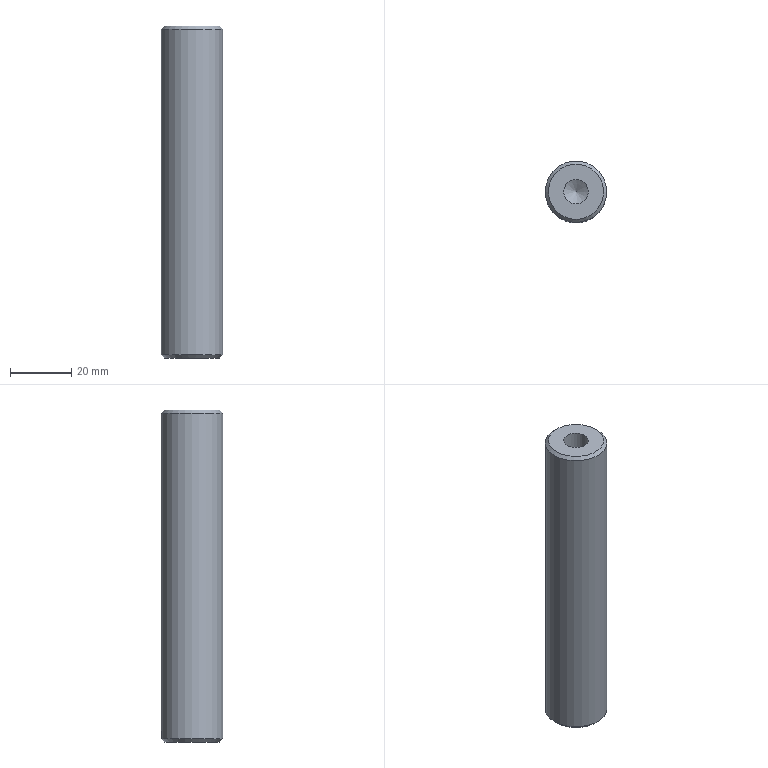Component | NX | GUIDE_POST | 1 solid | 9 faces | box 20 x 20 x 108 mm | volume 32179 mm3 | cone 4 | cylinder 3 | plane 2 | commonest cylinder face diameters 8 x2 20 x1
STEP:
#1=CARTESIAN_POINT('',(0.,0.,0.));
#2=DIRECTION('',(0.,0.,1.));
#3=DIRECTION('',(1.,0.,0.));
#4=AXIS2_PLACEMENT_3D('',#1,#2,#3);
#5=CARTESIAN_POINT('',(-177.087,-60.,105.));
#6=VERTEX_POINT('',#5);
#7=CARTESIAN_POINT('',(-186.087,-60.,105.));
#8=DIRECTION('',(0.,0.,1.));
#9=DIRECTION('',(1.,0.,0.));
#10=AXIS2_PLACEMENT_3D('',#7,#8,#9);
#11=CIRCLE('',#10,9.);
#12=CARTESIAN_POINT('',(-186.087,-60.,105.));
#13=DIRECTION('',(0.,0.,1.));
#14=DIRECTION('',(1.,0.,0.));
#15=AXIS2_PLACEMENT_3D('',#12,#13,#14);
#16=PLANE('',#15);
#17=CARTESIAN_POINT('',(0.,0.));
#18=DIRECTION('',(1.,0.));
#19=AXIS2_PLACEMENT_2D('',#17,#18);
#20=CIRCLE('',#19,9.);
#21=(GEOMETRIC_REPRESENTATION_CONTEXT(2)PARAMETRIC_REPRESENTATION_CONTEXT()REPRESENTATION_CONTEXT('',''));
#22=DEFINITIONAL_REPRESENTATION('',(#20),#21);
#23=PCURVE('',#16,#22);
#24=CARTESIAN_POINT('',(-186.087,-60.,104.));
#25=DIRECTION('',(0.,0.,-1.));
#26=DIRECTION('',(-1.,0.,0.));
#27=AXIS2_PLACEMENT_3D('',#24,#25,#26);
#28=CONICAL_SURFACE('',#27,10.,0.7854);
#29=CARTESIAN_POINT('',(9.425,-1.));
#30=DIRECTION('',(-1.,0.));
#31=VECTOR('',#30,1.);
#32=LINE('',#29,#31);
#33=(GEOMETRIC_REPRESENTATION_CONTEXT(2)PARAMETRIC_REPRESENTATION_CONTEXT()REPRESENTATION_CONTEXT('',''));
#34=DEFINITIONAL_REPRESENTATION('',(#32),#33);
#35=PCURVE('',#28,#34);
#36=SURFACE_CURVE('',#11,(#23,#35),.PCURVE_S1.);
#37=EDGE_CURVE('',#6,#6,#36,.T.);
#38=ORIENTED_EDGE('',*,*,#37,.T.);
#39=EDGE_LOOP('',(#38));
#40=FACE_BOUND('',#39,.T.);
#41=CARTESIAN_POINT('',(-190.087,-60.,105.));
#42=VERTEX_POINT('',#41);
#43=CARTESIAN_POINT('',(-186.087,-60.,105.));
#44=DIRECTION('',(0.,0.,-1.));
#45=DIRECTION('',(-1.,0.,0.));
#46=AXIS2_PLACEMENT_3D('',#43,#44,#45);
#47=CIRCLE('',#46,4.);
#48=CARTESIAN_POINT('',(-4.,0.));
#49=CARTESIAN_POINT('',(-4.,6.928));
#50=CARTESIAN_POINT('',(2.,3.464));
#51=CARTESIAN_POINT('',(8.,0.));
#52=CARTESIAN_POINT('',(2.,-3.464));
#53=CARTESIAN_POINT('',(-4.,-6.928));
#54=CARTESIAN_POINT('',(-4.,0.));
#55=(BOUNDED_CURVE()B_SPLINE_CURVE(2,(#48,#49,#50,#51,#52,#53,#54),.UNSPECIFIED.,.T.,.F.)B_SPLINE_CURVE_WITH_KNOTS((1,2,2,2,2,1),(-2.094,0.,2.094,4.189,6.283,8.378),.UNSPECIFIED.)CURVE()GEOMETRIC_REPRESENTATION_ITEM()RATIONAL_B_SPLINE_CURVE((1.,0.5,1.,0.5,1.,0.5,1.))REPRESENTATION_ITEM(''));
#56=(GEOMETRIC_REPRESENTATION_CONTEXT(2)PARAMETRIC_REPRESENTATION_CONTEXT()REPRESENTATION_CONTEXT('',''));
#57=DEFINITIONAL_REPRESENTATION('',(#55),#56);
#58=PCURVE('',#16,#57);
#59=CARTESIAN_POINT('',(-186.087,-60.,105.));
#60=DIRECTION('',(0.,0.,-1.));
#61=DIRECTION('',(-1.,0.,0.));
#62=AXIS2_PLACEMENT_3D('',#59,#60,#61);
#63=CYLINDRICAL_SURFACE('',#62,4.);
#64=CARTESIAN_POINT('',(0.,0.));
#65=DIRECTION('',(1.,0.));
#66=VECTOR('',#65,1.);
#67=LINE('',#64,#66);
#68=(GEOMETRIC_REPRESENTATION_CONTEXT(2)PARAMETRIC_REPRESENTATION_CONTEXT()REPRESENTATION_CONTEXT('',''));
#69=DEFINITIONAL_REPRESENTATION('',(#67),#68);
#70=PCURVE('',#63,#69);
#71=SURFACE_CURVE('',#47,(#58,#70),.PCURVE_S1.);
#72=EDGE_CURVE('',#42,#42,#71,.T.);
#73=ORIENTED_EDGE('',*,*,#72,.T.);
#74=EDGE_LOOP('',(#73));
#75=FACE_BOUND('',#74,.T.);
#76=ADVANCED_FACE('',(#40,#75),#16,.T.);
#77=CARTESIAN_POINT('',(-195.087,-60.,-3.));
#78=VERTEX_POINT('',#77);
#79=CARTESIAN_POINT('',(-186.087,-60.,-3.));
#80=DIRECTION('',(0.,0.,-1.));
#81=DIRECTION('',(-1.,0.,0.));
#82=AXIS2_PLACEMENT_3D('',#79,#80,#81);
#83=CIRCLE('',#82,9.);
#84=CARTESIAN_POINT('',(-186.087,-60.,-3.));
#85=DIRECTION('',(0.,0.,-1.));
#86=DIRECTION('',(-1.,0.,0.));
#87=AXIS2_PLACEMENT_3D('',#84,#85,#86);
#88=PLANE('',#87);
#89=CARTESIAN_POINT('',(0.,0.));
#90=DIRECTION('',(1.,0.));
#91=AXIS2_PLACEMENT_2D('',#89,#90);
#92=CIRCLE('',#91,9.);
#93=(GEOMETRIC_REPRESENTATION_CONTEXT(2)PARAMETRIC_REPRESENTATION_CONTEXT()REPRESENTATION_CONTEXT('',''));
#94=DEFINITIONAL_REPRESENTATION('',(#92),#93);
#95=PCURVE('',#88,#94);
#96=CARTESIAN_POINT('',(-186.087,-60.,-2.));
#97=DIRECTION('',(0.,0.,1.));
#98=DIRECTION('',(1.,0.,0.));
#99=AXIS2_PLACEMENT_3D('',#96,#97,#98);
#100=CONICAL_SURFACE('',#99,10.,0.7854);
#101=CARTESIAN_POINT('',(9.425,-1.));
#102=DIRECTION('',(-1.,0.));
#103=VECTOR('',#102,1.);
#104=LINE('',#101,#103);
#105=(GEOMETRIC_REPRESENTATION_CONTEXT(2)PARAMETRIC_REPRESENTATION_CONTEXT()REPRESENTATION_CONTEXT('',''));
#106=DEFINITIONAL_REPRESENTATION('',(#104),#105);
#107=PCURVE('',#100,#106);
#108=SURFACE_CURVE('',#83,(#95,#107),.PCURVE_S1.);
#109=EDGE_CURVE('',#78,#78,#108,.T.);
#110=ORIENTED_EDGE('',*,*,#109,.T.);
#111=EDGE_LOOP('',(#110));
#112=FACE_BOUND('',#111,.T.);
#113=CARTESIAN_POINT('',(-182.087,-60.,-3.));
#114=VERTEX_POINT('',#113);
#115=CARTESIAN_POINT('',(-186.087,-60.,-3.));
#116=DIRECTION('',(0.,0.,1.));
#117=DIRECTION('',(1.,0.,0.));
#118=AXIS2_PLACEMENT_3D('',#115,#116,#117);
#119=CIRCLE('',#118,4.);
#120=CARTESIAN_POINT('',(-4.,0.));
#121=CARTESIAN_POINT('',(-4.,6.928));
#122=CARTESIAN_POINT('',(2.,3.464));
#123=CARTESIAN_POINT('',(8.,0.));
#124=CARTESIAN_POINT('',(2.,-3.464));
#125=CARTESIAN_POINT('',(-4.,-6.928));
#126=CARTESIAN_POINT('',(-4.,0.));
#127=(BOUNDED_CURVE()B_SPLINE_CURVE(2,(#120,#121,#122,#123,#124,#125,#126),.UNSPECIFIED.,.T.,.F.)B_SPLINE_CURVE_WITH_KNOTS((1,2,2,2,2,1),(-2.094,0.,2.094,4.189,6.283,8.378),.UNSPECIFIED.)CURVE()GEOMETRIC_REPRESENTATION_ITEM()RATIONAL_B_SPLINE_CURVE((1.,0.5,1.,0.5,1.,0.5,1.))REPRESENTATION_ITEM(''));
#128=(GEOMETRIC_REPRESENTATION_CONTEXT(2)PARAMETRIC_REPRESENTATION_CONTEXT()REPRESENTATION_CONTEXT('',''));
#129=DEFINITIONAL_REPRESENTATION('',(#127),#128);
#130=PCURVE('',#88,#129);
#131=CARTESIAN_POINT('',(-186.087,-60.,-3.));
#132=DIRECTION('',(0.,0.,1.));
#133=DIRECTION('',(1.,0.,0.));
#134=AXIS2_PLACEMENT_3D('',#131,#132,#133);
#135=CYLINDRICAL_SURFACE('',#134,4.);
#136=CARTESIAN_POINT('',(0.,0.));
#137=DIRECTION('',(1.,0.));
#138=VECTOR('',#137,1.);
#139=LINE('',#136,#138);
#140=(GEOMETRIC_REPRESENTATION_CONTEXT(2)PARAMETRIC_REPRESENTATION_CONTEXT()REPRESENTATION_CONTEXT('',''));
#141=DEFINITIONAL_REPRESENTATION('',(#139),#140);
#142=PCURVE('',#135,#141);
#143=SURFACE_CURVE('',#119,(#130,#142),.PCURVE_S1.);
#144=EDGE_CURVE('',#114,#114,#143,.T.);
#145=ORIENTED_EDGE('',*,*,#144,.T.);
#146=EDGE_LOOP('',(#145));
#147=FACE_BOUND('',#146,.T.);
#148=ADVANCED_FACE('',(#112,#147),#88,.T.);
#149=CARTESIAN_POINT('',(-196.087,-60.,-2.));
#150=VERTEX_POINT('',#149);
#151=CARTESIAN_POINT('',(-176.087,-60.,-2.));
#152=VERTEX_POINT('',#151);
#153=CARTESIAN_POINT('',(-186.087,-60.,-2.));
#154=DIRECTION('',(0.,0.,1.));
#155=DIRECTION('',(-1.,0.,0.));
#156=AXIS2_PLACEMENT_3D('',#153,#154,#155);
#157=CIRCLE('',#156,10.);
#158=CARTESIAN_POINT('',(-186.087,-60.,-3.));
#159=DIRECTION('',(0.,0.,1.));
#160=DIRECTION('',(1.,0.,0.));
#161=AXIS2_PLACEMENT_3D('',#158,#159,#160);
#162=CYLINDRICAL_SURFACE('',#161,10.);
#163=CARTESIAN_POINT('',(3.142,1.));
#164=DIRECTION('',(1.,0.));
#165=VECTOR('',#164,1.);
#166=LINE('',#163,#165);
#167=(GEOMETRIC_REPRESENTATION_CONTEXT(2)PARAMETRIC_REPRESENTATION_CONTEXT()REPRESENTATION_CONTEXT('',''));
#168=DEFINITIONAL_REPRESENTATION('',(#166),#167);
#169=PCURVE('',#162,#168);
#170=CARTESIAN_POINT('',(3.142,0.));
#171=DIRECTION('',(1.,0.));
#172=VECTOR('',#171,1.);
#173=LINE('',#170,#172);
#174=(GEOMETRIC_REPRESENTATION_CONTEXT(2)PARAMETRIC_REPRESENTATION_CONTEXT()REPRESENTATION_CONTEXT('',''));
#175=DEFINITIONAL_REPRESENTATION('',(#173),#174);
#176=PCURVE('',#100,#175);
#177=SURFACE_CURVE('',#157,(#169,#176),.PCURVE_S1.);
#178=EDGE_CURVE('',#150,#152,#177,.T.);
#179=ORIENTED_EDGE('',*,*,#178,.T.);
#180=CARTESIAN_POINT('',(-176.087,-60.,104.));
#181=VERTEX_POINT('',#180);
#182=CARTESIAN_POINT('',(-176.087,-60.,-2.));
#183=CARTESIAN_POINT('',(-176.087,-60.,104.));
#184=B_SPLINE_CURVE_WITH_KNOTS('',1,(#182,#183),.UNSPECIFIED.,.F.,.F.,(2,2),(1.,107.),.PIECEWISE_BEZIER_KNOTS.);
#185=CARTESIAN_POINT('',(6.283,0.));
#186=DIRECTION('',(0.,1.));
#187=VECTOR('',#186,1.);
#188=LINE('',#185,#187);
#189=(GEOMETRIC_REPRESENTATION_CONTEXT(2)PARAMETRIC_REPRESENTATION_CONTEXT()REPRESENTATION_CONTEXT('',''));
#190=DEFINITIONAL_REPRESENTATION('',(#188),#189);
#191=PCURVE('',#162,#190);
#192=CARTESIAN_POINT('',(0.,0.));
#193=DIRECTION('',(0.,1.));
#194=VECTOR('',#193,1.);
#195=LINE('',#192,#194);
#196=(GEOMETRIC_REPRESENTATION_CONTEXT(2)PARAMETRIC_REPRESENTATION_CONTEXT()REPRESENTATION_CONTEXT('',''));
#197=DEFINITIONAL_REPRESENTATION('',(#195),#196);
#198=PCURVE('',#162,#197);
#199=SEAM_CURVE('',#184,(#191,#198),.PCURVE_S1.);
#200=EDGE_CURVE('',#152,#181,#199,.T.);
#201=ORIENTED_EDGE('',*,*,#200,.T.);
#202=CARTESIAN_POINT('',(-186.087,-60.,104.));
#203=DIRECTION('',(0.,0.,-1.));
#204=DIRECTION('',(1.,0.,0.));
#205=AXIS2_PLACEMENT_3D('',#202,#203,#204);
#206=CIRCLE('',#205,10.);
#207=CARTESIAN_POINT('',(6.283,107.));
#208=DIRECTION('',(-1.,0.));
#209=VECTOR('',#208,1.);
#210=LINE('',#207,#209);
#211=(GEOMETRIC_REPRESENTATION_CONTEXT(2)PARAMETRIC_REPRESENTATION_CONTEXT()REPRESENTATION_CONTEXT('',''));
#212=DEFINITIONAL_REPRESENTATION('',(#210),#211);
#213=PCURVE('',#162,#212);
#214=CARTESIAN_POINT('',(3.142,0.));
#215=DIRECTION('',(1.,0.));
#216=VECTOR('',#215,1.);
#217=LINE('',#214,#216);
#218=(GEOMETRIC_REPRESENTATION_CONTEXT(2)PARAMETRIC_REPRESENTATION_CONTEXT()REPRESENTATION_CONTEXT('',''));
#219=DEFINITIONAL_REPRESENTATION('',(#217),#218);
#220=PCURVE('',#28,#219);
#221=SURFACE_CURVE('',#206,(#213,#220),.PCURVE_S1.);
#222=EDGE_CURVE('',#181,#181,#221,.T.);
#223=ORIENTED_EDGE('',*,*,#222,.T.);
#224=ORIENTED_EDGE('',*,*,#200,.F.);
#225=CARTESIAN_POINT('',(-186.087,-60.,-2.));
#226=DIRECTION('',(0.,0.,1.));
#227=DIRECTION('',(-1.,0.,0.));
#228=AXIS2_PLACEMENT_3D('',#225,#226,#227);
#229=CIRCLE('',#228,10.);
#230=CARTESIAN_POINT('',(-3.142,1.));
#231=DIRECTION('',(1.,0.));
#232=VECTOR('',#231,1.);
#233=LINE('',#230,#232);
#234=(GEOMETRIC_REPRESENTATION_CONTEXT(2)PARAMETRIC_REPRESENTATION_CONTEXT()REPRESENTATION_CONTEXT('',''));
#235=DEFINITIONAL_REPRESENTATION('',(#233),#234);
#236=PCURVE('',#162,#235);
#237=CARTESIAN_POINT('',(3.142,0.));
#238=DIRECTION('',(1.,0.));
#239=VECTOR('',#238,1.);
#240=LINE('',#237,#239);
#241=(GEOMETRIC_REPRESENTATION_CONTEXT(2)PARAMETRIC_REPRESENTATION_CONTEXT()REPRESENTATION_CONTEXT('',''));
#242=DEFINITIONAL_REPRESENTATION('',(#240),#241);
#243=PCURVE('',#100,#242);
#244=SURFACE_CURVE('',#229,(#236,#243),.PCURVE_S1.);
#245=EDGE_CURVE('',#152,#150,#244,.T.);
#246=ORIENTED_EDGE('',*,*,#245,.T.);
#247=EDGE_LOOP('',(#179,#201,#223,#224,#246));
#248=FACE_BOUND('',#247,.T.);
#249=ADVANCED_FACE('',(#248),#162,.T.);
#250=CARTESIAN_POINT('',(-182.087,-60.,89.));
#251=VERTEX_POINT('',#250);
#252=CARTESIAN_POINT('',(-190.087,-60.,89.));
#253=VERTEX_POINT('',#252);
#254=CARTESIAN_POINT('',(-186.087,-60.,89.));
#255=DIRECTION('',(0.,0.,1.));
#256=DIRECTION('',(-1.,0.,0.));
#257=AXIS2_PLACEMENT_3D('',#254,#255,#256);
#258=CIRCLE('',#257,4.);
#259=CARTESIAN_POINT('',(-186.087,-60.,89.));
#260=DIRECTION('',(0.,0.,1.));
#261=DIRECTION('',(1.,0.,0.));
#262=AXIS2_PLACEMENT_3D('',#259,#260,#261);
#263=CONICAL_SURFACE('',#262,4.,1.03);
#264=CARTESIAN_POINT('',(-3.142,0.));
#265=DIRECTION('',(1.,0.));
#266=VECTOR('',#265,1.);
#267=LINE('',#264,#266);
#268=(GEOMETRIC_REPRESENTATION_CONTEXT(2)PARAMETRIC_REPRESENTATION_CONTEXT()REPRESENTATION_CONTEXT('',''));
#269=DEFINITIONAL_REPRESENTATION('',(#267),#268);
#270=PCURVE('',#263,#269);
#271=CARTESIAN_POINT('',(6.283,16.));
#272=DIRECTION('',(-1.,0.));
#273=VECTOR('',#272,1.);
#274=LINE('',#271,#273);
#275=(GEOMETRIC_REPRESENTATION_CONTEXT(2)PARAMETRIC_REPRESENTATION_CONTEXT()REPRESENTATION_CONTEXT('',''));
#276=DEFINITIONAL_REPRESENTATION('',(#274),#275);
#277=PCURVE('',#63,#276);
#278=SURFACE_CURVE('',#258,(#270,#277),.PCURVE_S1.);
#279=EDGE_CURVE('',#251,#253,#278,.T.);
#280=ORIENTED_EDGE('',*,*,#279,.F.);
#281=CARTESIAN_POINT('',(-186.087,-60.,86.597));
#282=VERTEX_POINT('',#281);
#283=CARTESIAN_POINT('',(-186.087,-60.,86.597));
#284=CARTESIAN_POINT('',(-182.087,-60.,89.));
#285=B_SPLINE_CURVE_WITH_KNOTS('',1,(#283,#284),.UNSPECIFIED.,.F.,.F.,(2,2),(-4.667,0.),.PIECEWISE_BEZIER_KNOTS.);
#286=CARTESIAN_POINT('',(0.,0.));
#287=DIRECTION('',(0.,1.));
#288=VECTOR('',#287,1.);
#289=LINE('',#286,#288);
#290=(GEOMETRIC_REPRESENTATION_CONTEXT(2)PARAMETRIC_REPRESENTATION_CONTEXT()REPRESENTATION_CONTEXT('',''));
#291=DEFINITIONAL_REPRESENTATION('',(#289),#290);
#292=PCURVE('',#263,#291);
#293=CARTESIAN_POINT('',(6.283,0.));
#294=DIRECTION('',(0.,1.));
#295=VECTOR('',#294,1.);
#296=LINE('',#293,#295);
#297=(GEOMETRIC_REPRESENTATION_CONTEXT(2)PARAMETRIC_REPRESENTATION_CONTEXT()REPRESENTATION_CONTEXT('',''));
#298=DEFINITIONAL_REPRESENTATION('',(#296),#297);
#299=PCURVE('',#263,#298);
#300=SEAM_CURVE('',#285,(#292,#299),.PCURVE_S1.);
#301=EDGE_CURVE('',#282,#251,#300,.T.);
#302=ORIENTED_EDGE('',*,*,#301,.F.);
#303=ORIENTED_EDGE('',*,*,#301,.T.);
#304=CARTESIAN_POINT('',(-186.087,-60.,89.));
#305=DIRECTION('',(0.,0.,1.));
#306=DIRECTION('',(-1.,0.,0.));
#307=AXIS2_PLACEMENT_3D('',#304,#305,#306);
#308=CIRCLE('',#307,4.);
#309=CARTESIAN_POINT('',(3.142,0.));
#310=DIRECTION('',(1.,0.));
#311=VECTOR('',#310,1.);
#312=LINE('',#309,#311);
#313=(GEOMETRIC_REPRESENTATION_CONTEXT(2)PARAMETRIC_REPRESENTATION_CONTEXT()REPRESENTATION_CONTEXT('',''));
#314=DEFINITIONAL_REPRESENTATION('',(#312),#313);
#315=PCURVE('',#263,#314);
#316=CARTESIAN_POINT('',(6.283,16.));
#317=DIRECTION('',(-1.,0.));
#318=VECTOR('',#317,1.);
#319=LINE('',#316,#318);
#320=(GEOMETRIC_REPRESENTATION_CONTEXT(2)PARAMETRIC_REPRESENTATION_CONTEXT()REPRESENTATION_CONTEXT('',''));
#321=DEFINITIONAL_REPRESENTATION('',(#319),#320);
#322=PCURVE('',#63,#321);
#323=SURFACE_CURVE('',#308,(#315,#322),.PCURVE_S1.);
#324=EDGE_CURVE('',#253,#251,#323,.T.);
#325=ORIENTED_EDGE('',*,*,#324,.F.);
#326=EDGE_LOOP('',(#280,#302,#303,#325));
#327=FACE_BOUND('',#326,.F.);
#328=ADVANCED_FACE('',(#327),#263,.F.);
#329=ORIENTED_EDGE('',*,*,#279,.T.);
#330=CARTESIAN_POINT('',(-190.087,-60.,105.));
#331=CARTESIAN_POINT('',(-190.087,-60.,89.));
#332=B_SPLINE_CURVE_WITH_KNOTS('',1,(#330,#331),.UNSPECIFIED.,.F.,.F.,(2,2),(0.,16.),.PIECEWISE_BEZIER_KNOTS.);
#333=CARTESIAN_POINT('',(0.,0.));
#334=DIRECTION('',(0.,1.));
#335=VECTOR('',#334,1.);
#336=LINE('',#333,#335);
#337=(GEOMETRIC_REPRESENTATION_CONTEXT(2)PARAMETRIC_REPRESENTATION_CONTEXT()REPRESENTATION_CONTEXT('',''));
#338=DEFINITIONAL_REPRESENTATION('',(#336),#337);
#339=PCURVE('',#63,#338);
#340=CARTESIAN_POINT('',(6.283,0.));
#341=DIRECTION('',(0.,1.));
#342=VECTOR('',#341,1.);
#343=LINE('',#340,#342);
#344=(GEOMETRIC_REPRESENTATION_CONTEXT(2)PARAMETRIC_REPRESENTATION_CONTEXT()REPRESENTATION_CONTEXT('',''));
#345=DEFINITIONAL_REPRESENTATION('',(#343),#344);
#346=PCURVE('',#63,#345);
#347=SEAM_CURVE('',#332,(#339,#346),.PCURVE_S1.);
#348=EDGE_CURVE('',#42,#253,#347,.T.);
#349=ORIENTED_EDGE('',*,*,#348,.F.);
#350=ORIENTED_EDGE('',*,*,#72,.T.);
#351=ORIENTED_EDGE('',*,*,#348,.T.);
#352=ORIENTED_EDGE('',*,*,#324,.T.);
#353=EDGE_LOOP('',(#329,#349,#350,#351,#352));
#354=FACE_BOUND('',#353,.F.);
#355=ADVANCED_FACE('',(#354),#63,.F.);
#356=CARTESIAN_POINT('',(-190.087,-60.,13.));
#357=VERTEX_POINT('',#356);
#358=CARTESIAN_POINT('',(-182.087,-60.,13.));
#359=VERTEX_POINT('',#358);
#360=CARTESIAN_POINT('',(-186.087,-60.,13.));
#361=DIRECTION('',(0.,0.,-1.));
#362=DIRECTION('',(1.,0.,0.));
#363=AXIS2_PLACEMENT_3D('',#360,#361,#362);
#364=CIRCLE('',#363,4.);
#365=CARTESIAN_POINT('',(-186.087,-60.,13.));
#366=DIRECTION('',(0.,0.,-1.));
#367=DIRECTION('',(-1.,0.,0.));
#368=AXIS2_PLACEMENT_3D('',#365,#366,#367);
#369=CONICAL_SURFACE('',#368,4.,1.03);
#370=CARTESIAN_POINT('',(-3.142,0.));
#371=DIRECTION('',(1.,0.));
#372=VECTOR('',#371,1.);
#373=LINE('',#370,#372);
#374=(GEOMETRIC_REPRESENTATION_CONTEXT(2)PARAMETRIC_REPRESENTATION_CONTEXT()REPRESENTATION_CONTEXT('',''));
#375=DEFINITIONAL_REPRESENTATION('',(#373),#374);
#376=PCURVE('',#369,#375);
#377=CARTESIAN_POINT('',(6.283,16.));
#378=DIRECTION('',(-1.,0.));
#379=VECTOR('',#378,1.);
#380=LINE('',#377,#379);
#381=(GEOMETRIC_REPRESENTATION_CONTEXT(2)PARAMETRIC_REPRESENTATION_CONTEXT()REPRESENTATION_CONTEXT('',''));
#382=DEFINITIONAL_REPRESENTATION('',(#380),#381);
#383=PCURVE('',#135,#382);
#384=SURFACE_CURVE('',#364,(#376,#383),.PCURVE_S1.);
#385=EDGE_CURVE('',#357,#359,#384,.T.);
#386=ORIENTED_EDGE('',*,*,#385,.F.);
#387=CARTESIAN_POINT('',(-186.087,-60.,15.403));
#388=VERTEX_POINT('',#387);
#389=CARTESIAN_POINT('',(-186.087,-60.,15.403));
#390=CARTESIAN_POINT('',(-190.087,-60.,13.));
#391=B_SPLINE_CURVE_WITH_KNOTS('',1,(#389,#390),.UNSPECIFIED.,.F.,.F.,(2,2),(-4.667,0.),.PIECEWISE_BEZIER_KNOTS.);
#392=CARTESIAN_POINT('',(0.,0.));
#393=DIRECTION('',(0.,1.));
#394=VECTOR('',#393,1.);
#395=LINE('',#392,#394);
#396=(GEOMETRIC_REPRESENTATION_CONTEXT(2)PARAMETRIC_REPRESENTATION_CONTEXT()REPRESENTATION_CONTEXT('',''));
#397=DEFINITIONAL_REPRESENTATION('',(#395),#396);
#398=PCURVE('',#369,#397);
#399=CARTESIAN_POINT('',(6.283,0.));
#400=DIRECTION('',(0.,1.));
#401=VECTOR('',#400,1.);
#402=LINE('',#399,#401);
#403=(GEOMETRIC_REPRESENTATION_CONTEXT(2)PARAMETRIC_REPRESENTATION_CONTEXT()REPRESENTATION_CONTEXT('',''));
#404=DEFINITIONAL_REPRESENTATION('',(#402),#403);
#405=PCURVE('',#369,#404);
#406=SEAM_CURVE('',#391,(#398,#405),.PCURVE_S1.);
#407=EDGE_CURVE('',#388,#357,#406,.T.);
#408=ORIENTED_EDGE('',*,*,#407,.F.);
#409=ORIENTED_EDGE('',*,*,#407,.T.);
#410=CARTESIAN_POINT('',(-186.087,-60.,13.));
#411=DIRECTION('',(0.,0.,-1.));
#412=DIRECTION('',(1.,0.,0.));
#413=AXIS2_PLACEMENT_3D('',#410,#411,#412);
#414=CIRCLE('',#413,4.);
#415=CARTESIAN_POINT('',(3.142,0.));
#416=DIRECTION('',(1.,0.));
#417=VECTOR('',#416,1.);
#418=LINE('',#415,#417);
#419=(GEOMETRIC_REPRESENTATION_CONTEXT(2)PARAMETRIC_REPRESENTATION_CONTEXT()REPRESENTATION_CONTEXT('',''));
#420=DEFINITIONAL_REPRESENTATION('',(#418),#419);
#421=PCURVE('',#369,#420);
#422=CARTESIAN_POINT('',(6.283,16.));
#423=DIRECTION('',(-1.,0.));
#424=VECTOR('',#423,1.);
#425=LINE('',#422,#424);
#426=(GEOMETRIC_REPRESENTATION_CONTEXT(2)PARAMETRIC_REPRESENTATION_CONTEXT()REPRESENTATION_CONTEXT('',''));
#427=DEFINITIONAL_REPRESENTATION('',(#425),#426);
#428=PCURVE('',#135,#427);
#429=SURFACE_CURVE('',#414,(#421,#428),.PCURVE_S1.);
#430=EDGE_CURVE('',#359,#357,#429,.T.);
#431=ORIENTED_EDGE('',*,*,#430,.F.);
#432=EDGE_LOOP('',(#386,#408,#409,#431));
#433=FACE_BOUND('',#432,.F.);
#434=ADVANCED_FACE('',(#433),#369,.F.);
#435=ORIENTED_EDGE('',*,*,#385,.T.);
#436=CARTESIAN_POINT('',(-182.087,-60.,-3.));
#437=CARTESIAN_POINT('',(-182.087,-60.,13.));
#438=B_SPLINE_CURVE_WITH_KNOTS('',1,(#436,#437),.UNSPECIFIED.,.F.,.F.,(2,2),(0.,16.),.PIECEWISE_BEZIER_KNOTS.);
#439=CARTESIAN_POINT('',(0.,0.));
#440=DIRECTION('',(0.,1.));
#441=VECTOR('',#440,1.);
#442=LINE('',#439,#441);
#443=(GEOMETRIC_REPRESENTATION_CONTEXT(2)PARAMETRIC_REPRESENTATION_CONTEXT()REPRESENTATION_CONTEXT('',''));
#444=DEFINITIONAL_REPRESENTATION('',(#442),#443);
#445=PCURVE('',#135,#444);
#446=CARTESIAN_POINT('',(6.283,0.));
#447=DIRECTION('',(0.,1.));
#448=VECTOR('',#447,1.);
#449=LINE('',#446,#448);
#450=(GEOMETRIC_REPRESENTATION_CONTEXT(2)PARAMETRIC_REPRESENTATION_CONTEXT()REPRESENTATION_CONTEXT('',''));
#451=DEFINITIONAL_REPRESENTATION('',(#449),#450);
#452=PCURVE('',#135,#451);
#453=SEAM_CURVE('',#438,(#445,#452),.PCURVE_S1.);
#454=EDGE_CURVE('',#114,#359,#453,.T.);
#455=ORIENTED_EDGE('',*,*,#454,.F.);
#456=ORIENTED_EDGE('',*,*,#144,.T.);
#457=ORIENTED_EDGE('',*,*,#454,.T.);
#458=ORIENTED_EDGE('',*,*,#430,.T.);
#459=EDGE_LOOP('',(#435,#455,#456,#457,#458));
#460=FACE_BOUND('',#459,.F.);
#461=ADVANCED_FACE('',(#460),#135,.F.);
#462=ORIENTED_EDGE('',*,*,#109,.F.);
#463=CARTESIAN_POINT('',(-195.087,-60.,-3.));
#464=CARTESIAN_POINT('',(-196.087,-60.,-2.));
#465=B_SPLINE_CURVE_WITH_KNOTS('',1,(#463,#464),.UNSPECIFIED.,.F.,.F.,(2,2),(-1.414,0.),.PIECEWISE_BEZIER_KNOTS.);
#466=CARTESIAN_POINT('',(9.425,0.));
#467=DIRECTION('',(0.,1.));
#468=VECTOR('',#467,1.);
#469=LINE('',#466,#468);
#470=(GEOMETRIC_REPRESENTATION_CONTEXT(2)PARAMETRIC_REPRESENTATION_CONTEXT()REPRESENTATION_CONTEXT('',''));
#471=DEFINITIONAL_REPRESENTATION('',(#469),#470);
#472=PCURVE('',#100,#471);
#473=CARTESIAN_POINT('',(3.142,0.));
#474=DIRECTION('',(0.,1.));
#475=VECTOR('',#474,1.);
#476=LINE('',#473,#475);
#477=(GEOMETRIC_REPRESENTATION_CONTEXT(2)PARAMETRIC_REPRESENTATION_CONTEXT()REPRESENTATION_CONTEXT('',''));
#478=DEFINITIONAL_REPRESENTATION('',(#476),#477);
#479=PCURVE('',#100,#478);
#480=SEAM_CURVE('',#465,(#472,#479),.PCURVE_S1.);
#481=EDGE_CURVE('',#78,#150,#480,.T.);
#482=ORIENTED_EDGE('',*,*,#481,.T.);
#483=ORIENTED_EDGE('',*,*,#245,.F.);
#484=ORIENTED_EDGE('',*,*,#178,.F.);
#485=ORIENTED_EDGE('',*,*,#481,.F.);
#486=EDGE_LOOP('',(#462,#482,#483,#484,#485));
#487=FACE_BOUND('',#486,.T.);
#488=ADVANCED_FACE('',(#487),#100,.T.);
#489=ORIENTED_EDGE('',*,*,#37,.F.);
#490=CARTESIAN_POINT('',(-177.087,-60.,105.));
#491=CARTESIAN_POINT('',(-176.087,-60.,104.));
#492=B_SPLINE_CURVE_WITH_KNOTS('',1,(#490,#491),.UNSPECIFIED.,.F.,.F.,(2,2),(-1.414,0.),.PIECEWISE_BEZIER_KNOTS.);
#493=CARTESIAN_POINT('',(9.425,0.));
#494=DIRECTION('',(0.,1.));
#495=VECTOR('',#494,1.);
#496=LINE('',#493,#495);
#497=(GEOMETRIC_REPRESENTATION_CONTEXT(2)PARAMETRIC_REPRESENTATION_CONTEXT()REPRESENTATION_CONTEXT('',''));
#498=DEFINITIONAL_REPRESENTATION('',(#496),#497);
#499=PCURVE('',#28,#498);
#500=CARTESIAN_POINT('',(3.142,0.));
#501=DIRECTION('',(0.,1.));
#502=VECTOR('',#501,1.);
#503=LINE('',#500,#502);
#504=(GEOMETRIC_REPRESENTATION_CONTEXT(2)PARAMETRIC_REPRESENTATION_CONTEXT()REPRESENTATION_CONTEXT('',''));
#505=DEFINITIONAL_REPRESENTATION('',(#503),#504);
#506=PCURVE('',#28,#505);
#507=SEAM_CURVE('',#492,(#499,#506),.PCURVE_S1.);
#508=EDGE_CURVE('',#6,#181,#507,.T.);
#509=ORIENTED_EDGE('',*,*,#508,.T.);
#510=ORIENTED_EDGE('',*,*,#222,.F.);
#511=ORIENTED_EDGE('',*,*,#508,.F.);
#512=EDGE_LOOP('',(#489,#509,#510,#511));
#513=FACE_BOUND('',#512,.T.);
#514=ADVANCED_FACE('',(#513),#28,.T.);
#515=CLOSED_SHELL('',(#76,#148,#249,#328,#355,#434,#461,#488,#514));
#516=MANIFOLD_SOLID_BREP('',#515);
#517=(LENGTH_UNIT()NAMED_UNIT(*)SI_UNIT(.MILLI.,.METRE.));
#518=UNCERTAINTY_MEASURE_WITH_UNIT(LENGTH_MEASURE(0.00001),#517,'','');
#519=(NAMED_UNIT(*)PLANE_ANGLE_UNIT()SI_UNIT($,.RADIAN.));
#520=(NAMED_UNIT(*)SI_UNIT($,.STERADIAN.)SOLID_ANGLE_UNIT());
#521=(GEOMETRIC_REPRESENTATION_CONTEXT(3)GLOBAL_UNCERTAINTY_ASSIGNED_CONTEXT((#518))GLOBAL_UNIT_ASSIGNED_CONTEXT((#517,#519,#520))REPRESENTATION_CONTEXT('',''));
#522=ADVANCED_BREP_SHAPE_REPRESENTATION('',(#4,#516),#521);